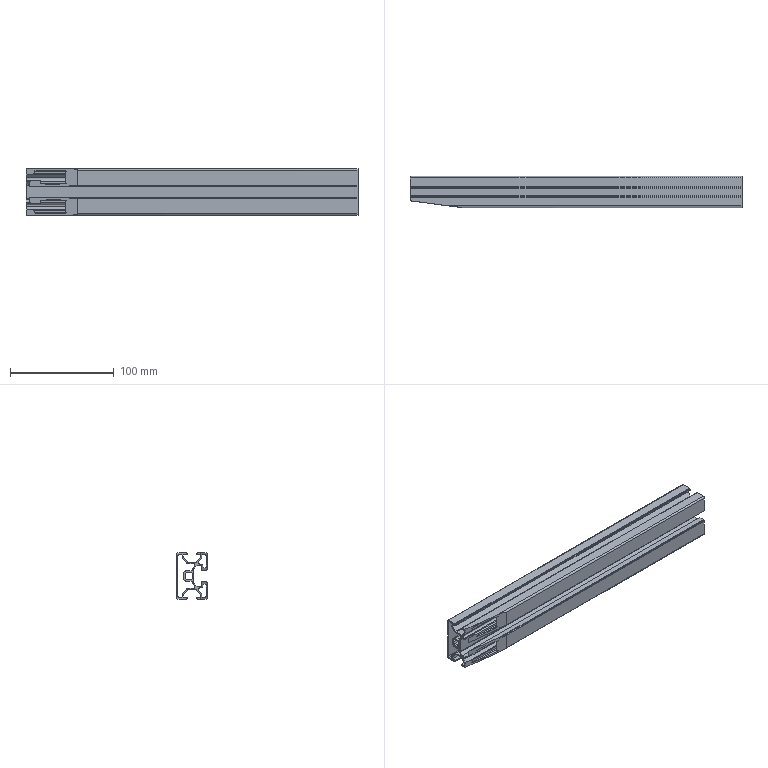Component | SolidWorks | 170423A4-AOB02-H3045M-L320-1 | 1 solid | 134 faces | volume 119352 mm3 | plane 88 | cylinder 46 | commonest cylinder face diameters 2 x27 3 x8 6.8 x5 8.5 x4 5 x2